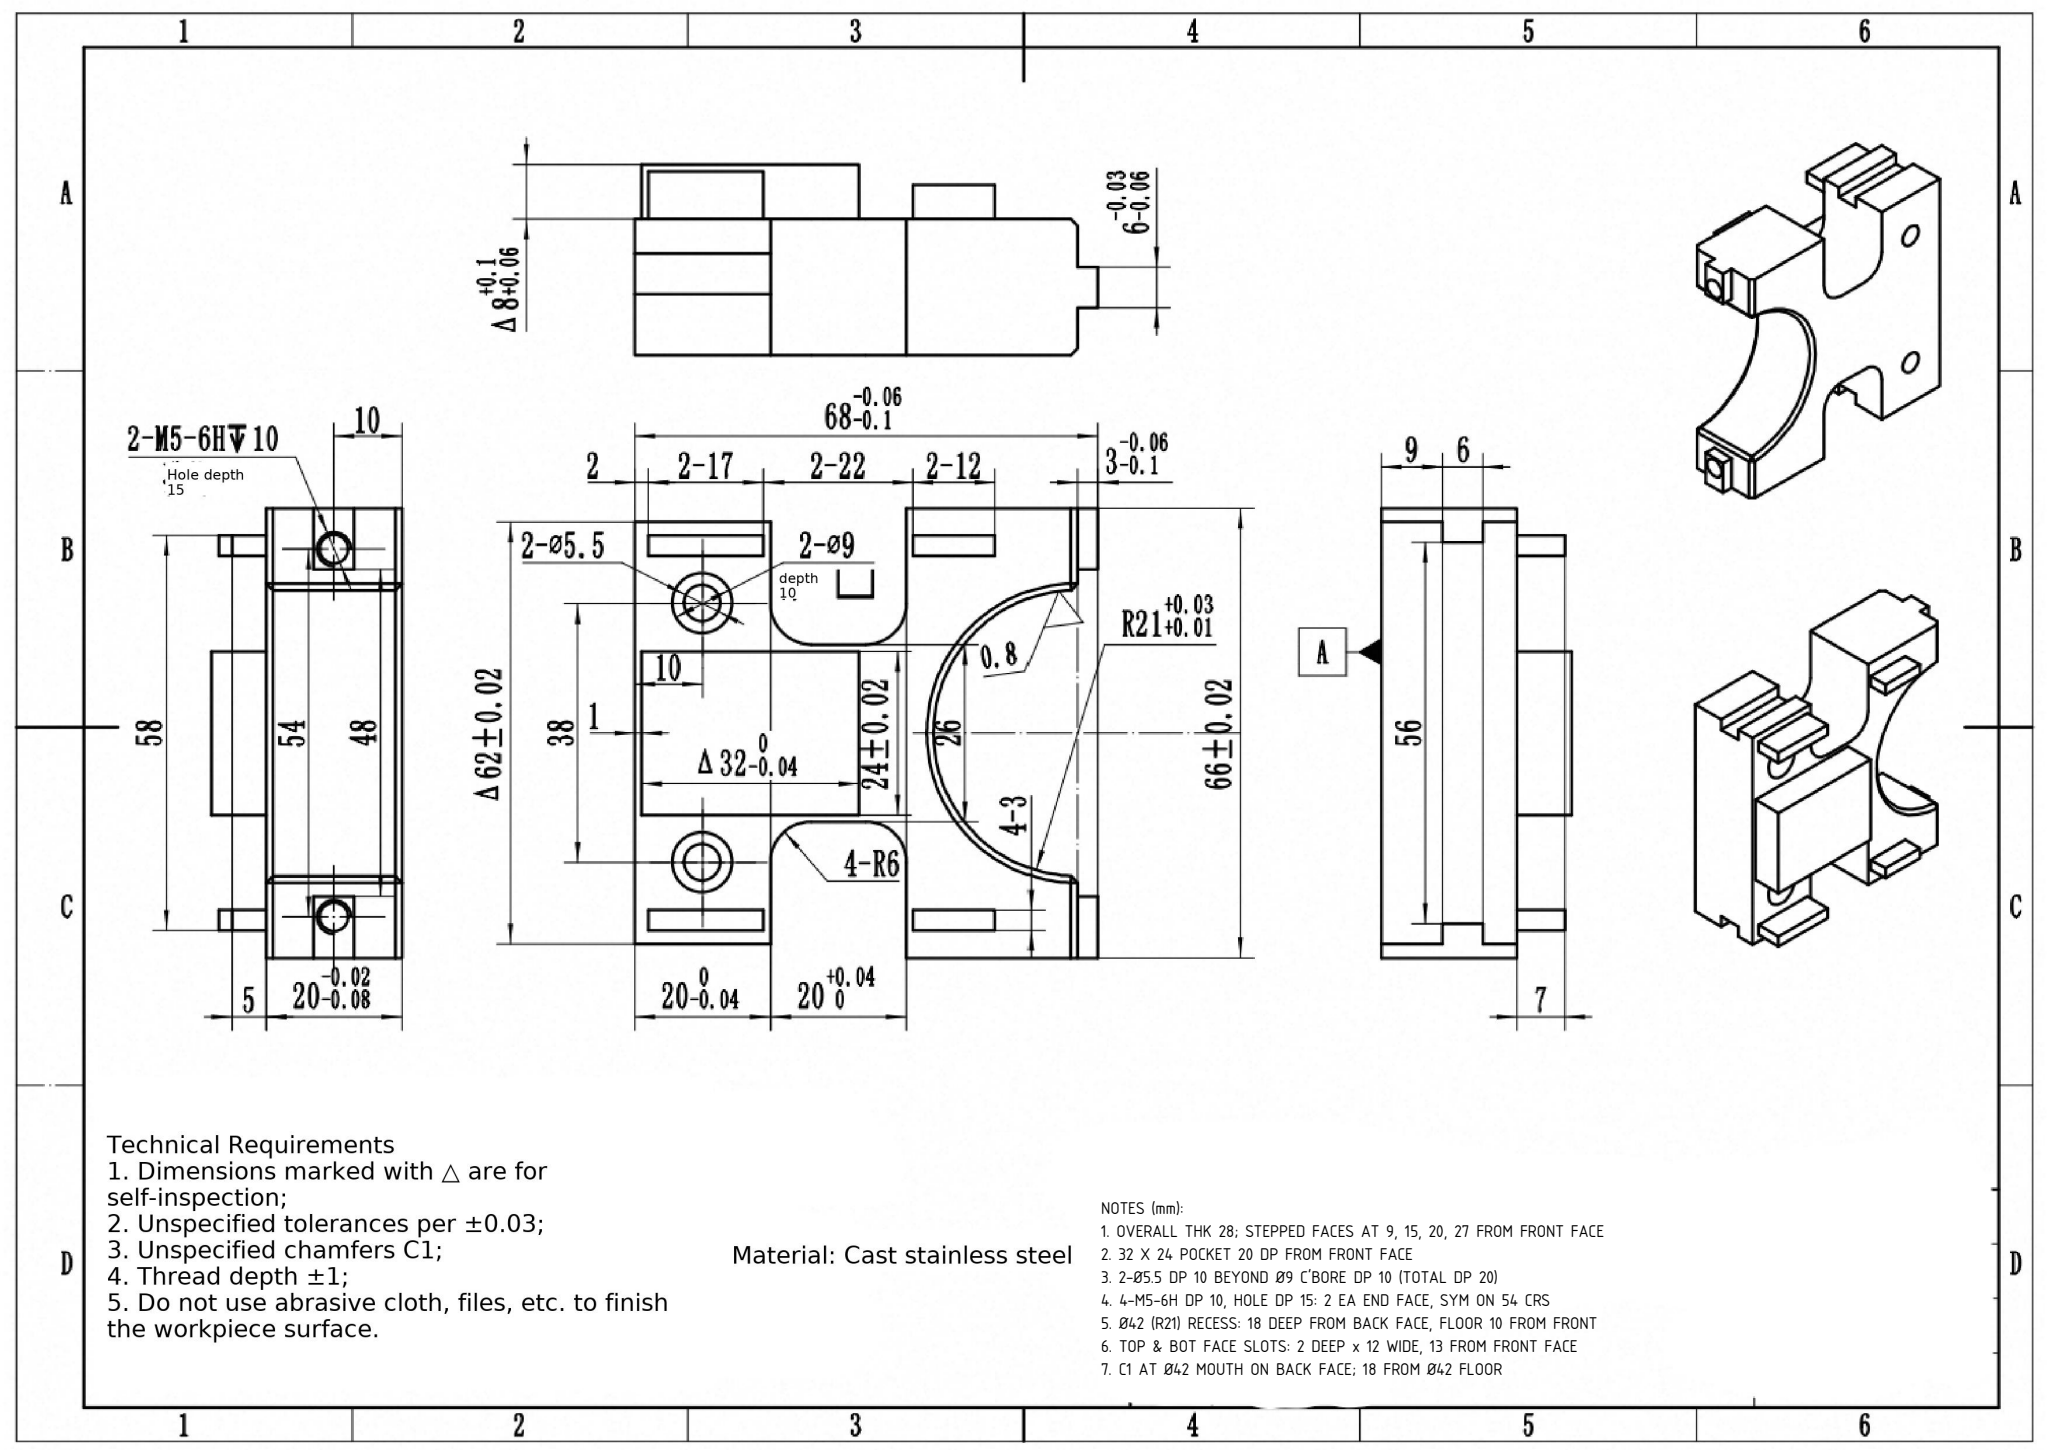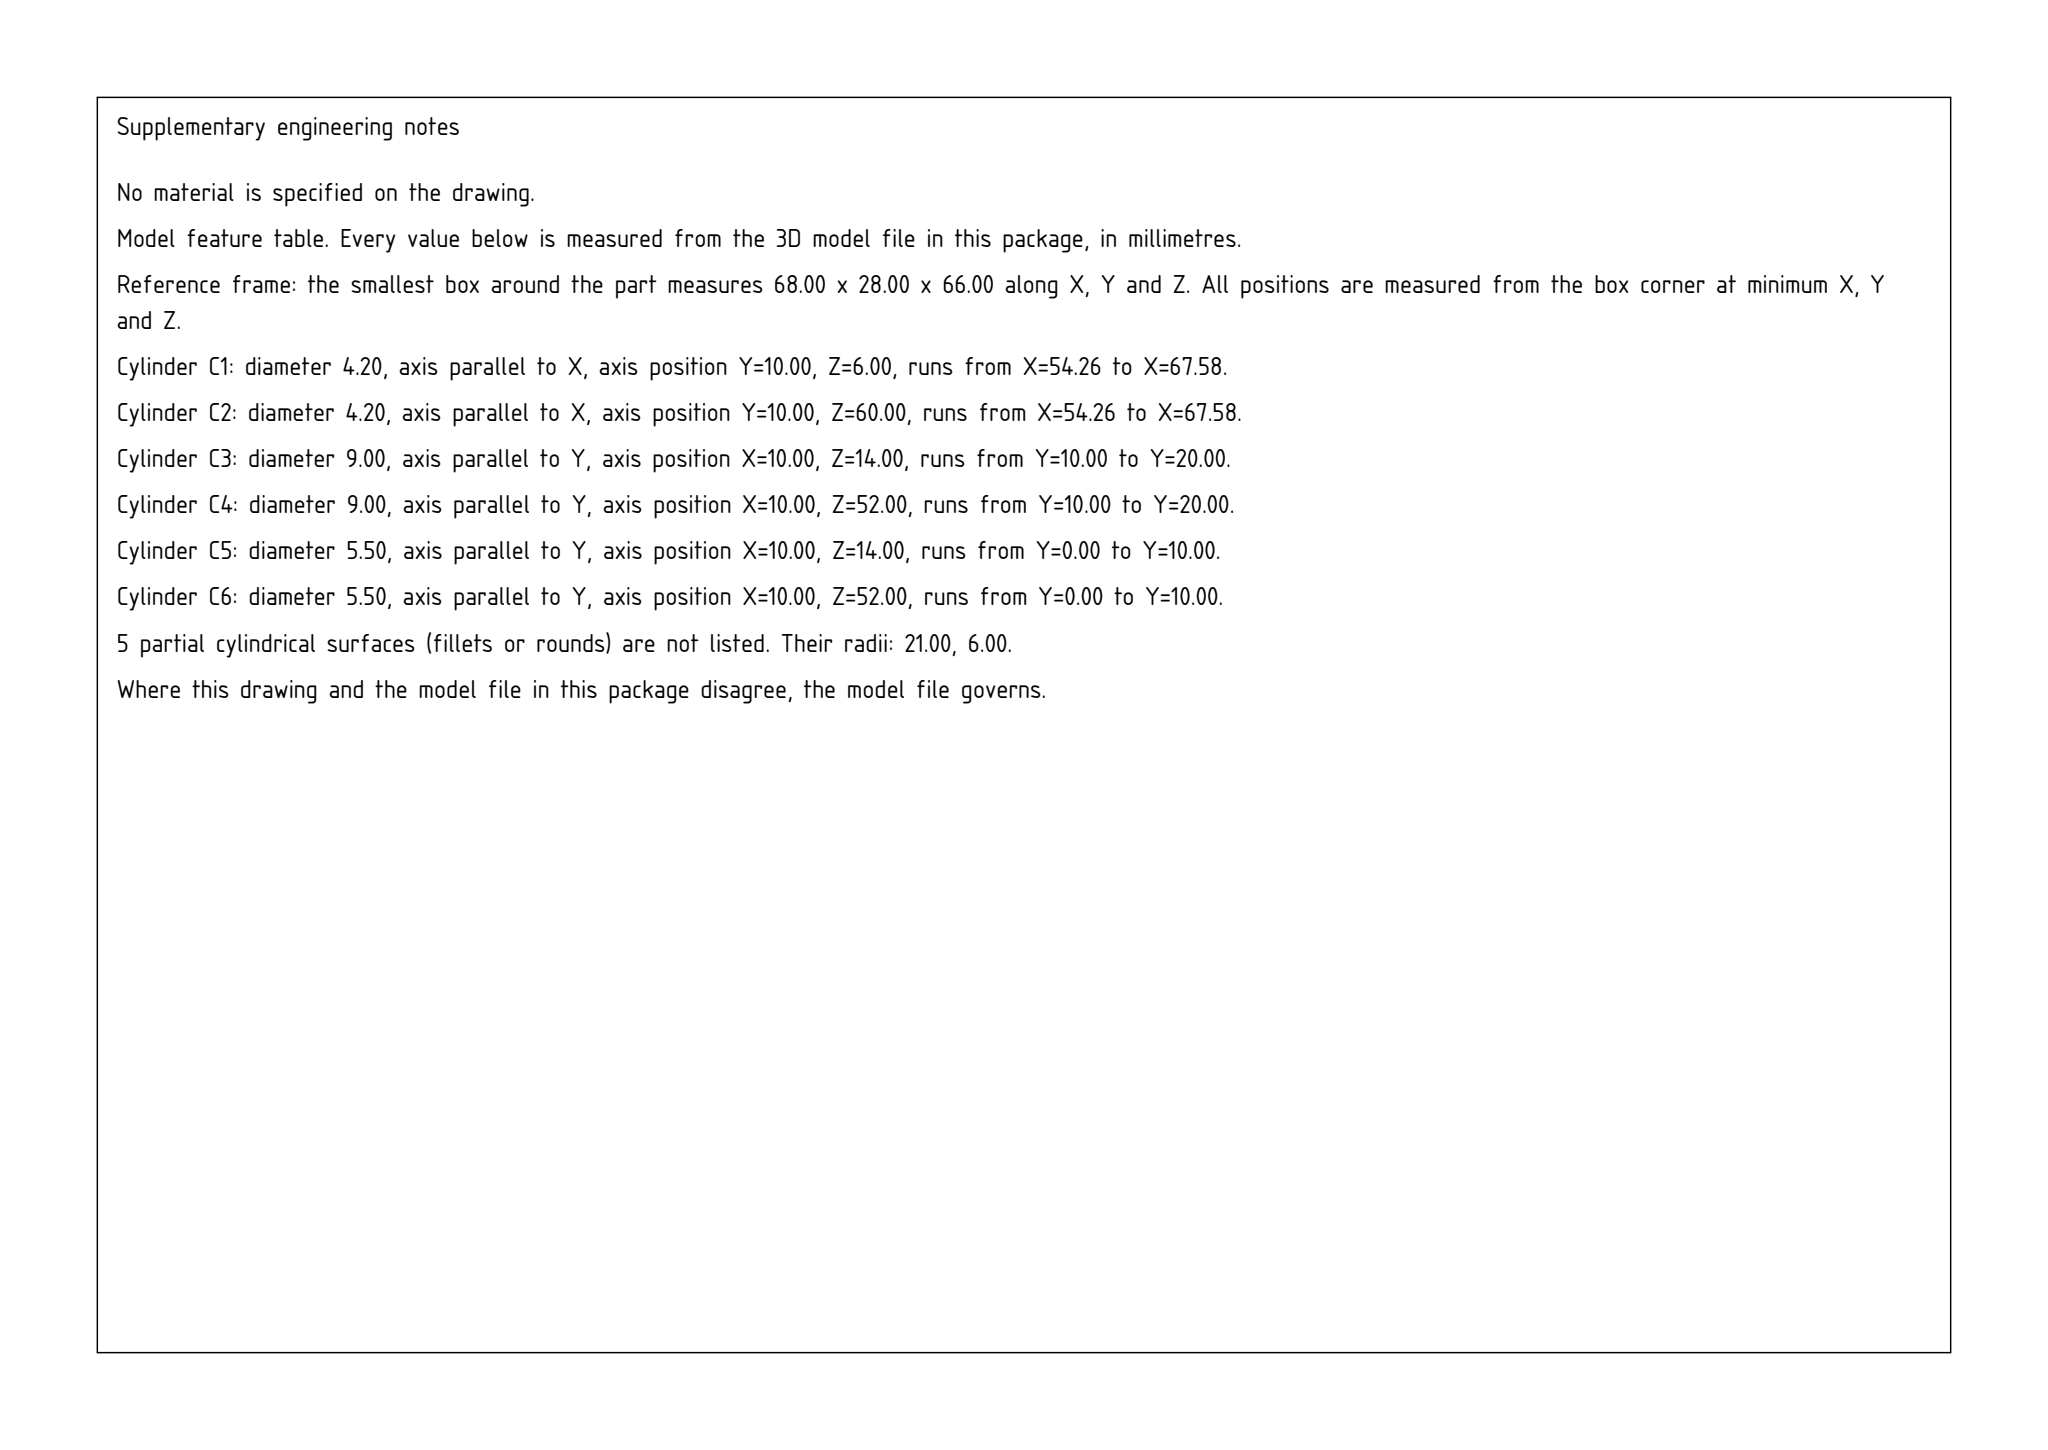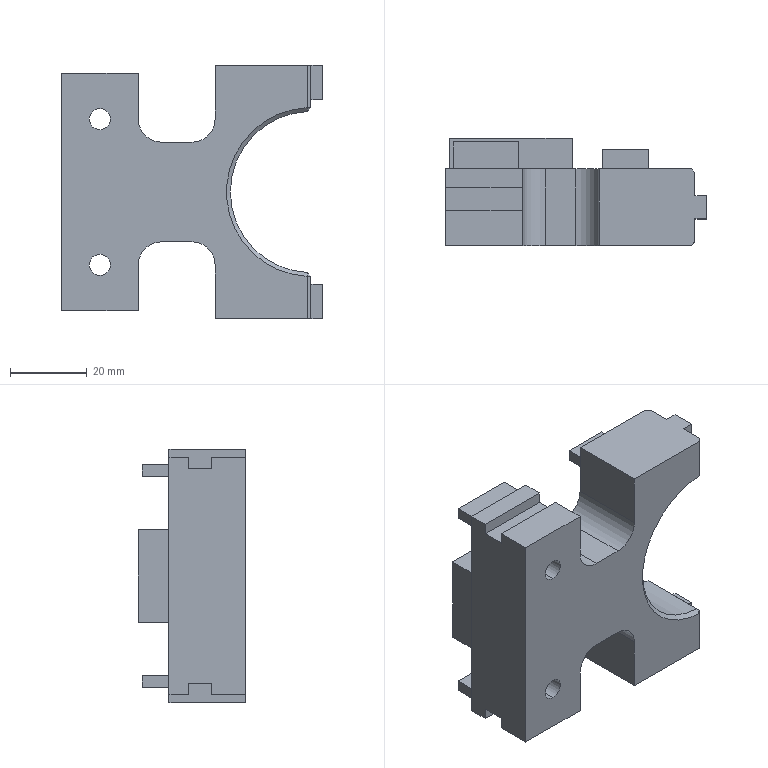Part | SolidWorks | mm | 1 solid | 95 faces | box 68 x 28 x 66 mm | volume 59536 mm3 | plane 68 | cylinder 17 | cone 10 | commonest cylinder face diameters 4.2 x4 9 x4 5.5 x4 12 x4 42 x1
Drawing notes:
OVERALL THK 28; STEPPED FACES AT 9, 15, 20, 27 FROM FRONT FACE | from the solid: Y-normal planes at 0,9,15,20,27,28; bbox Y = 28.0
32 X 24 POCKET 20 DP FROM FRONT FACE | from the solid: Pocket walls x=1..33 (32), z=21..45 (24); floor plane y=20.0 from front face y=0
2-Ø5.5 DP 10 BEYOND Ø9 C'BORE DP 10 (TOTAL DP 20) | from the solid: cyl Ø5.5 axis y len 10 at (x10,z14)&(x10,z52); coaxial Ø9 axis y len 10 same positions
4-M5-6H DP 10, HOLE DP 15: 2 EA END FACE, SYM ON 54 CRS | from the solid: 4x Ø4.2 tap-drill cyls axis x, len 13.31, at (y10,z6) & (y10,z60), 2 ea; z6/z60 = 54 apart, sym about z33 of 66 height; planes x0 & x68 end faces
Ø42 (R21) RECESS: 18 DEEP FROM BACK FACE, FLOOR 10 FROM FRONT | from the solid: cyl dia 42 axis y at x=65,z=33, len 18; y-planes 10 & 28 (bbox y=28)
TOP & BOT FACE SLOTS: 2 DEEP x 12 WIDE, 13 FROM FRONT FACE | from the solid: z-planes 64 & 2 (2 from top/bot faces 66/0); y-planes 13 & 25 = 12 wide
C1 AT Ø42 MOUTH ON BACK FACE; 18 FROM Ø42 FLOOR | from the solid: cones 90 deg ref dia 42/44 at open end y=28; Ø42 floor at y=10